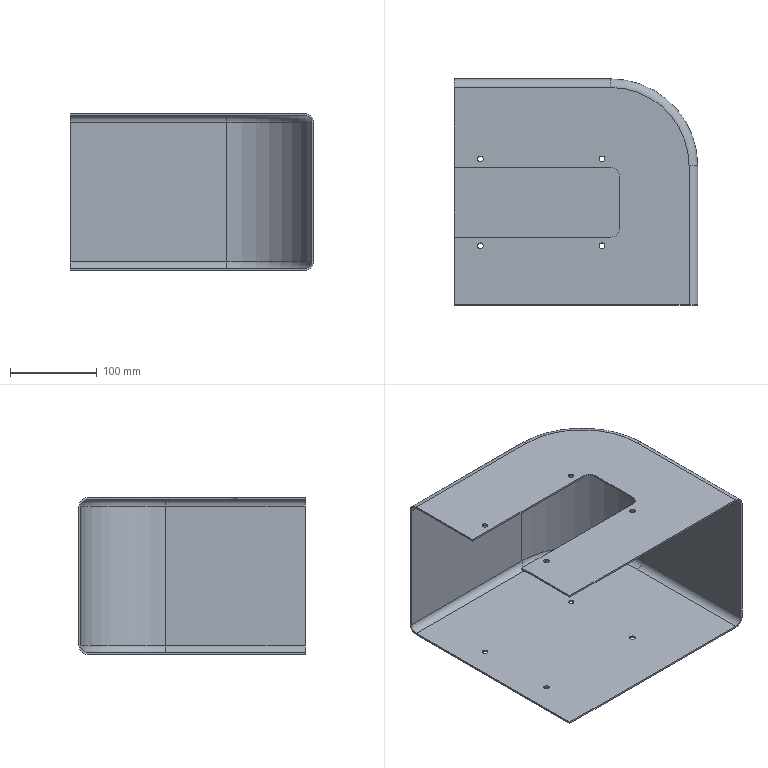Component | SolidWorks | WT-FLD-EJG-1212-00-023-1 | 1 solid | 46 faces | box 280 x 260 x 180 mm | volume 418497 mm3 | cylinder 28 | plane 14 | torus 4 | commonest cylinder face diameters 6.5 x16 20 x6 16 x4 200 x1 196 x1 | material AISI 1045 Steel, cold drawn
build123d program:
from build123d import *

# Parameters (mm, degrees)
BOSS_EXTRUDE1_DEPTH        = 90
FILLET1_R                  = 10
SHELL1_T                   = -2
CUT_EXTRUDE2_REACH         = 424.374
F_6_5_6_5_DIAMETER_HOLE1_D = 6.5


with BuildPart() as part:
    # Sketch1 → Boss-Extrude1 (new, symmetric)
    with BuildSketch(Plane.XY):
        with BuildLine():
            Line((0, 0), (-280, 0))
            Line((-280, 0), (-280, 160))
            ThreePointArc((-280, 160), (-250.711, 230.711), (-180, 260))
            Line((-180, 260), (0, 260))
            Line((0, 260), (0, 0))
        make_face()
    extrude(amount=BOSS_EXTRUDE1_DEPTH, both=True)

    # Fillet1
    fillet1_edges = [part.edges().sort_by_distance(p)[0] for p in [
        (-250.711, 230.711, 90),
        (-280, 80, 90),
        (-280, 80, -90),
        (-250.711, 230.711, -90),
        (-90, 260, -90),
        (-90, 260, 90),
    ]]
    fillet(fillet1_edges, radius=FILLET1_R)

    # Shell1
    shell1_openings = [part.faces().sort_by_distance(p)[0] for p in [
        (0, 129.883, 0),
        (-139.883, 0, 0),
    ]]
    offset(amount=SHELL1_T, openings=shell1_openings, kind=Kind.INTERSECTION)

    # Sketch3 → Cut-Extrude2 (cut, up to next)
    with BuildSketch(Plane(origin=(0, 0, -90), x_dir=(-1, 0, 0), z_dir=(0, 0, -1)), mode=Mode.PRIVATE) as cut_extrude2_sk1:
        with BuildLine():
            Line((180, 158), (0, 158))
            Line((0, 158), (0, 78))
            Line((0, 78), (180, 78))
            ThreePointArc((180, 78), (187.071, 80.929), (190, 88))
            Line((190, 88), (190, 148))
            ThreePointArc((190, 148), (187.071, 155.071), (180, 158))
        make_face()
    cut_extrude2_tool1 = extrude(cut_extrude2_sk1.sketch, amount=-CUT_EXTRUDE2_REACH, mode=Mode.PRIVATE) & part.part
    add(cut_extrude2_tool1.solids().sort_by_distance((-94.737, 118, -90))[0], mode=Mode.SUBTRACT)

    # 6.5 _6.5_ Diameter Hole1 (through all)
    with Locations(Plane(origin=(0, 0, -90), x_dir=(-1, 0, 0), z_dir=(0, 0, -1))):
        with Locations((30, 168), (30, 68), (170, 68), (170, 168)):
            Hole(F_6_5_6_5_DIAMETER_HOLE1_D / 2)


solid = part.part

# Placed as in the assembly
solid = solid.moved(Location((-127, -118, 0), (-180, 0, 180)))